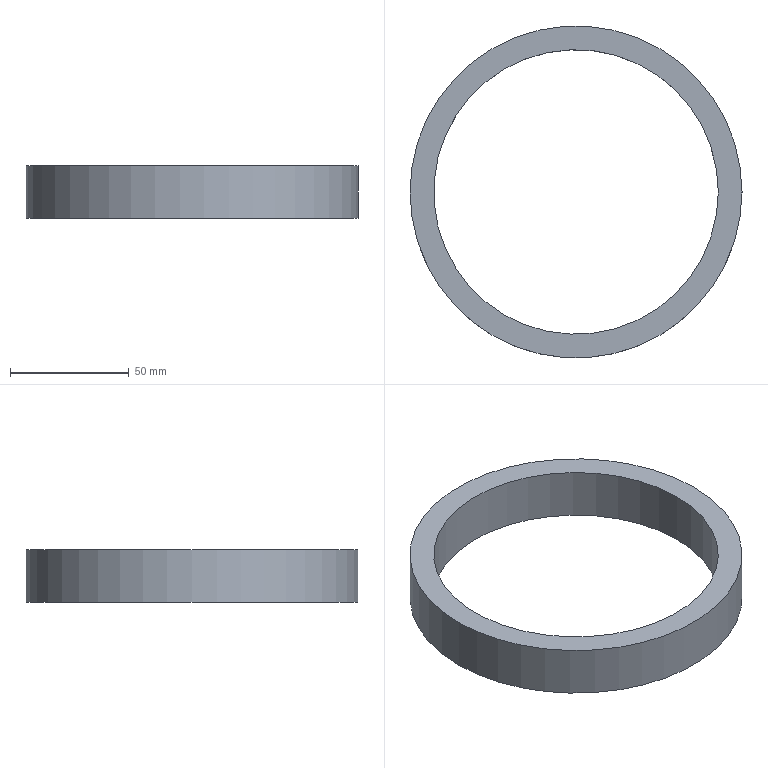Component | NX | CH3404-6 | 1 solid | 4 faces | box 140 x 140 x 22 mm | volume 89850 mm3 | cylinder 2 | plane 2 | commonest cylinder face diameters 140 x1 120 x1
STEP:
#1=CARTESIAN_POINT('',(0.,0.,0.));
#2=DIRECTION('',(0.,0.,1.));
#3=DIRECTION('',(1.,0.,0.));
#4=AXIS2_PLACEMENT_3D('',#1,#2,#3);
#5=CARTESIAN_POINT('',(70.531,0.1057,-1470.003));
#6=VERTEX_POINT('',#5);
#7=CARTESIAN_POINT('',(0.5308,0.1057,-1470.003));
#8=DIRECTION('',(0.,0.,1.));
#9=DIRECTION('',(1.,0.,0.));
#10=AXIS2_PLACEMENT_3D('',#7,#8,#9);
#11=CIRCLE('',#10,70.);
#12=CARTESIAN_POINT('',(0.5308,0.1057,-1470.003));
#13=DIRECTION('',(0.,0.,-1.));
#14=DIRECTION('',(-1.,0.,0.));
#15=AXIS2_PLACEMENT_3D('',#12,#13,#14);
#16=CYLINDRICAL_SURFACE('',#15,70.);
#17=CARTESIAN_POINT('',(9.425,0.));
#18=DIRECTION('',(-1.,0.));
#19=VECTOR('',#18,1.);
#20=LINE('',#17,#19);
#21=(GEOMETRIC_REPRESENTATION_CONTEXT(2)PARAMETRIC_REPRESENTATION_CONTEXT()REPRESENTATION_CONTEXT('',''));
#22=DEFINITIONAL_REPRESENTATION('',(#20),#21);
#23=PCURVE('',#16,#22);
#24=CARTESIAN_POINT('',(0.5308,0.1057,-1470.003));
#25=DIRECTION('',(0.,0.,1.));
#26=DIRECTION('',(1.,0.,0.));
#27=AXIS2_PLACEMENT_3D('',#24,#25,#26);
#28=PLANE('',#27);
#29=CARTESIAN_POINT('',(0.,0.));
#30=DIRECTION('',(1.,0.));
#31=AXIS2_PLACEMENT_2D('',#29,#30);
#32=CIRCLE('',#31,70.);
#33=(GEOMETRIC_REPRESENTATION_CONTEXT(2)PARAMETRIC_REPRESENTATION_CONTEXT()REPRESENTATION_CONTEXT('',''));
#34=DEFINITIONAL_REPRESENTATION('',(#32),#33);
#35=PCURVE('',#28,#34);
#36=SURFACE_CURVE('',#11,(#23,#35),.PCURVE_S1.);
#37=EDGE_CURVE('',#6,#6,#36,.T.);
#38=ORIENTED_EDGE('',*,*,#37,.F.);
#39=CARTESIAN_POINT('',(70.531,0.1057,-1492.003));
#40=VERTEX_POINT('',#39);
#41=CARTESIAN_POINT('',(70.531,0.1057,-1470.003));
#42=CARTESIAN_POINT('',(70.531,0.1057,-1492.003));
#43=B_SPLINE_CURVE_WITH_KNOTS('',1,(#41,#42),.UNSPECIFIED.,.F.,.F.,(2,2),(0.,22.),.PIECEWISE_BEZIER_KNOTS.);
#44=CARTESIAN_POINT('',(9.425,0.));
#45=DIRECTION('',(0.,1.));
#46=VECTOR('',#45,1.);
#47=LINE('',#44,#46);
#48=(GEOMETRIC_REPRESENTATION_CONTEXT(2)PARAMETRIC_REPRESENTATION_CONTEXT()REPRESENTATION_CONTEXT('',''));
#49=DEFINITIONAL_REPRESENTATION('',(#47),#48);
#50=PCURVE('',#16,#49);
#51=CARTESIAN_POINT('',(3.142,0.));
#52=DIRECTION('',(0.,1.));
#53=VECTOR('',#52,1.);
#54=LINE('',#51,#53);
#55=(GEOMETRIC_REPRESENTATION_CONTEXT(2)PARAMETRIC_REPRESENTATION_CONTEXT()REPRESENTATION_CONTEXT('',''));
#56=DEFINITIONAL_REPRESENTATION('',(#54),#55);
#57=PCURVE('',#16,#56);
#58=SEAM_CURVE('',#43,(#50,#57),.PCURVE_S1.);
#59=EDGE_CURVE('',#6,#40,#58,.T.);
#60=ORIENTED_EDGE('',*,*,#59,.T.);
#61=CARTESIAN_POINT('',(0.5308,0.1057,-1492.003));
#62=DIRECTION('',(0.,0.,1.));
#63=DIRECTION('',(1.,0.,0.));
#64=AXIS2_PLACEMENT_3D('',#61,#62,#63);
#65=CIRCLE('',#64,70.);
#66=CARTESIAN_POINT('',(9.425,22.));
#67=DIRECTION('',(-1.,0.));
#68=VECTOR('',#67,1.);
#69=LINE('',#66,#68);
#70=(GEOMETRIC_REPRESENTATION_CONTEXT(2)PARAMETRIC_REPRESENTATION_CONTEXT()REPRESENTATION_CONTEXT('',''));
#71=DEFINITIONAL_REPRESENTATION('',(#69),#70);
#72=PCURVE('',#16,#71);
#73=CARTESIAN_POINT('',(0.5308,0.1057,-1492.003));
#74=DIRECTION('',(0.,0.,1.));
#75=DIRECTION('',(1.,0.,0.));
#76=AXIS2_PLACEMENT_3D('',#73,#74,#75);
#77=PLANE('',#76);
#78=CARTESIAN_POINT('',(0.,0.));
#79=DIRECTION('',(1.,0.));
#80=AXIS2_PLACEMENT_2D('',#78,#79);
#81=CIRCLE('',#80,70.);
#82=(GEOMETRIC_REPRESENTATION_CONTEXT(2)PARAMETRIC_REPRESENTATION_CONTEXT()REPRESENTATION_CONTEXT('',''));
#83=DEFINITIONAL_REPRESENTATION('',(#81),#82);
#84=PCURVE('',#77,#83);
#85=SURFACE_CURVE('',#65,(#72,#84),.PCURVE_S1.);
#86=EDGE_CURVE('',#40,#40,#85,.T.);
#87=ORIENTED_EDGE('',*,*,#86,.T.);
#88=ORIENTED_EDGE('',*,*,#59,.F.);
#89=EDGE_LOOP('',(#38,#60,#87,#88));
#90=FACE_BOUND('',#89,.T.);
#91=ADVANCED_FACE('',(#90),#16,.T.);
#92=CARTESIAN_POINT('',(60.531,0.1057,-1470.003));
#93=VERTEX_POINT('',#92);
#94=CARTESIAN_POINT('',(0.5308,0.1057,-1470.003));
#95=DIRECTION('',(0.,0.,1.));
#96=DIRECTION('',(1.,0.,0.));
#97=AXIS2_PLACEMENT_3D('',#94,#95,#96);
#98=CIRCLE('',#97,60.);
#99=CARTESIAN_POINT('',(0.5308,0.1057,-1470.003));
#100=DIRECTION('',(0.,0.,-1.));
#101=DIRECTION('',(-1.,0.,0.));
#102=AXIS2_PLACEMENT_3D('',#99,#100,#101);
#103=CYLINDRICAL_SURFACE('',#102,60.);
#104=CARTESIAN_POINT('',(9.425,0.));
#105=DIRECTION('',(-1.,0.));
#106=VECTOR('',#105,1.);
#107=LINE('',#104,#106);
#108=(GEOMETRIC_REPRESENTATION_CONTEXT(2)PARAMETRIC_REPRESENTATION_CONTEXT()REPRESENTATION_CONTEXT('',''));
#109=DEFINITIONAL_REPRESENTATION('',(#107),#108);
#110=PCURVE('',#103,#109);
#111=CARTESIAN_POINT('',(0.,0.));
#112=DIRECTION('',(1.,0.));
#113=AXIS2_PLACEMENT_2D('',#111,#112);
#114=CIRCLE('',#113,60.);
#115=(GEOMETRIC_REPRESENTATION_CONTEXT(2)PARAMETRIC_REPRESENTATION_CONTEXT()REPRESENTATION_CONTEXT('',''));
#116=DEFINITIONAL_REPRESENTATION('',(#114),#115);
#117=PCURVE('',#28,#116);
#118=SURFACE_CURVE('',#98,(#110,#117),.PCURVE_S1.);
#119=EDGE_CURVE('',#93,#93,#118,.T.);
#120=ORIENTED_EDGE('',*,*,#119,.F.);
#121=CARTESIAN_POINT('',(60.531,0.1057,-1492.003));
#122=VERTEX_POINT('',#121);
#123=CARTESIAN_POINT('',(60.531,0.1057,-1470.003));
#124=CARTESIAN_POINT('',(60.531,0.1057,-1492.003));
#125=B_SPLINE_CURVE_WITH_KNOTS('',1,(#123,#124),.UNSPECIFIED.,.F.,.F.,(2,2),(0.,22.),.PIECEWISE_BEZIER_KNOTS.);
#126=CARTESIAN_POINT('',(9.425,0.));
#127=DIRECTION('',(0.,1.));
#128=VECTOR('',#127,1.);
#129=LINE('',#126,#128);
#130=(GEOMETRIC_REPRESENTATION_CONTEXT(2)PARAMETRIC_REPRESENTATION_CONTEXT()REPRESENTATION_CONTEXT('',''));
#131=DEFINITIONAL_REPRESENTATION('',(#129),#130);
#132=PCURVE('',#103,#131);
#133=CARTESIAN_POINT('',(3.142,0.));
#134=DIRECTION('',(0.,1.));
#135=VECTOR('',#134,1.);
#136=LINE('',#133,#135);
#137=(GEOMETRIC_REPRESENTATION_CONTEXT(2)PARAMETRIC_REPRESENTATION_CONTEXT()REPRESENTATION_CONTEXT('',''));
#138=DEFINITIONAL_REPRESENTATION('',(#136),#137);
#139=PCURVE('',#103,#138);
#140=SEAM_CURVE('',#125,(#132,#139),.PCURVE_S1.);
#141=EDGE_CURVE('',#93,#122,#140,.T.);
#142=ORIENTED_EDGE('',*,*,#141,.T.);
#143=CARTESIAN_POINT('',(0.5308,0.1057,-1492.003));
#144=DIRECTION('',(0.,0.,1.));
#145=DIRECTION('',(1.,0.,0.));
#146=AXIS2_PLACEMENT_3D('',#143,#144,#145);
#147=CIRCLE('',#146,60.);
#148=CARTESIAN_POINT('',(9.425,22.));
#149=DIRECTION('',(-1.,0.));
#150=VECTOR('',#149,1.);
#151=LINE('',#148,#150);
#152=(GEOMETRIC_REPRESENTATION_CONTEXT(2)PARAMETRIC_REPRESENTATION_CONTEXT()REPRESENTATION_CONTEXT('',''));
#153=DEFINITIONAL_REPRESENTATION('',(#151),#152);
#154=PCURVE('',#103,#153);
#155=CARTESIAN_POINT('',(0.,0.));
#156=DIRECTION('',(1.,0.));
#157=AXIS2_PLACEMENT_2D('',#155,#156);
#158=CIRCLE('',#157,60.);
#159=(GEOMETRIC_REPRESENTATION_CONTEXT(2)PARAMETRIC_REPRESENTATION_CONTEXT()REPRESENTATION_CONTEXT('',''));
#160=DEFINITIONAL_REPRESENTATION('',(#158),#159);
#161=PCURVE('',#77,#160);
#162=SURFACE_CURVE('',#147,(#154,#161),.PCURVE_S1.);
#163=EDGE_CURVE('',#122,#122,#162,.T.);
#164=ORIENTED_EDGE('',*,*,#163,.T.);
#165=ORIENTED_EDGE('',*,*,#141,.F.);
#166=EDGE_LOOP('',(#120,#142,#164,#165));
#167=FACE_BOUND('',#166,.F.);
#168=ADVANCED_FACE('',(#167),#103,.F.);
#169=ORIENTED_EDGE('',*,*,#37,.T.);
#170=EDGE_LOOP('',(#169));
#171=FACE_BOUND('',#170,.T.);
#172=ORIENTED_EDGE('',*,*,#119,.F.);
#173=EDGE_LOOP('',(#172));
#174=FACE_BOUND('',#173,.T.);
#175=ADVANCED_FACE('',(#171,#174),#28,.T.);
#176=ORIENTED_EDGE('',*,*,#86,.F.);
#177=EDGE_LOOP('',(#176));
#178=FACE_BOUND('',#177,.T.);
#179=ORIENTED_EDGE('',*,*,#163,.T.);
#180=EDGE_LOOP('',(#179));
#181=FACE_BOUND('',#180,.T.);
#182=ADVANCED_FACE('',(#178,#181),#77,.F.);
#183=CLOSED_SHELL('',(#91,#168,#175,#182));
#184=MANIFOLD_SOLID_BREP('',#183);
#185=(LENGTH_UNIT()NAMED_UNIT(*)SI_UNIT(.MILLI.,.METRE.));
#186=UNCERTAINTY_MEASURE_WITH_UNIT(LENGTH_MEASURE(0.00001),#185,'','');
#187=(NAMED_UNIT(*)PLANE_ANGLE_UNIT()SI_UNIT($,.RADIAN.));
#188=(NAMED_UNIT(*)SI_UNIT($,.STERADIAN.)SOLID_ANGLE_UNIT());
#189=(GEOMETRIC_REPRESENTATION_CONTEXT(3)GLOBAL_UNCERTAINTY_ASSIGNED_CONTEXT((#186))GLOBAL_UNIT_ASSIGNED_CONTEXT((#185,#187,#188))REPRESENTATION_CONTEXT('',''));
#190=ADVANCED_BREP_SHAPE_REPRESENTATION('',(#4,#184),#189);